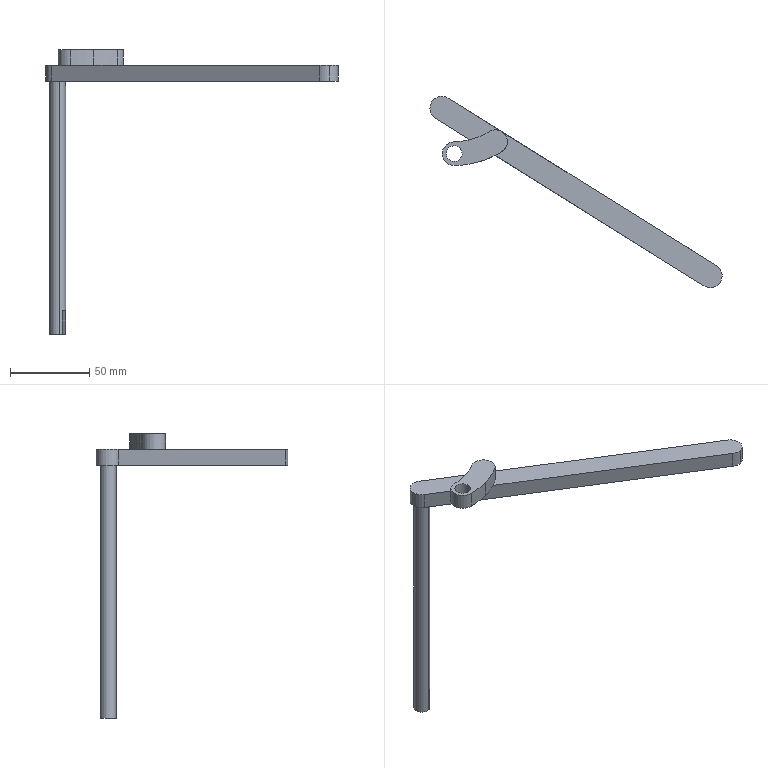Component | SolidWorks | DRocker(Right)-1 | 1 solid | 31 faces | box 184.66 x 120.91 x 180 mm | volume 48377 mm3 | cylinder 17 | plane 14 | commonest cylinder face diameters 15 x5 7 x4 10 x4 120 x2 90 x2
build123d program:
from build123d import *

# Parameters (mm, degrees)
BOSS_EXTRUDE1_DEPTH = 10
SKETCH1_3_R         = 5
BOSS_EXTRUDE2_DEPTH = 160
BOSS_EXTRUDE3_START = 10
SKETCH1_4_2_R       = 5
BOSS_EXTRUDE3_DEPTH = 10
SKETCH2_R           = 5
BOSS_EXTRUDE4_DEPTH = 10
CUT_EXTRUDE1_DEPTH  = 15
SKETCH4_R           = 3.5
CUT_EXTRUDE2_DEPTH  = 10


with BuildPart() as part:
    # Sketch1_4 → Boss-Extrude1 (new body)
    with BuildSketch(Plane.XY):
        with BuildLine():
            Line((-210.677, 89.978), (-358.098, -45.177))
            ThreePointArc((-358.098, -45.177), (-368.695, -44.717), (-368.235, -34.121))
            Line((-368.235, -34.121), (-220.814, 101.035))
            ThreePointArc((-220.814, 101.035), (-210.217, 100.575), (-210.677, 89.978))
        make_face()
    extrude(amount=BOSS_EXTRUDE1_DEPTH)

    # Sketch1_3 → Boss-Extrude2 (add)
    with BuildSketch(Plane.XY):
        with Locations((-215.746, 95.507)):
            Circle(SKETCH1_3_R)
    extrude(amount=-BOSS_EXTRUDE2_DEPTH)

    # Sketch1_4 2 → Boss-Extrude3 (add)
    with BuildSketch(Plane.XY.offset(BOSS_EXTRUDE3_START)):
        with Locations((-245.23, 68.476)):
            Circle(SKETCH1_4_2_R)
    extrude(amount=BOSS_EXTRUDE3_DEPTH)

    # Sketch2 → Boss-Extrude4 (add)
    with BuildSketch(Plane.XY.offset(10)):
        with BuildLine():
            ThreePointArc((-252.451, 66.449), (-254.679, 81.953), (-252.818, 97.505))
            ThreePointArc((-252.818, 97.505), (-243.695, 102.917), (-238.284, 93.794))
            ThreePointArc((-238.284, 93.794), (-239.68, 82.13), (-238.009, 70.502))
            ThreePointArc((-238.009, 70.502), (-243.203, 61.255), (-252.451, 66.449))
        make_face()
        with Locations(Location((-245.551, 95.65, 0), (0, 0, 180))):
            Circle(SKETCH2_R, mode=Mode.SUBTRACT)
    extrude(amount=BOSS_EXTRUDE4_DEPTH)

    # Sketch3 → Cut-Extrude1 (cut)
    with BuildSketch(Plane(origin=(0, 0, -160), x_dir=(-1, 0, 0), z_dir=(0, 0, -1))):
        Polygon((214.394, 94.033), (221.765, 87.275), (224.468, 90.223), (217.097, 96.981), align=None)
    extrude(amount=-CUT_EXTRUDE1_DEPTH, mode=Mode.SUBTRACT)

    # Sketch4 → Cut-Extrude2 (cut)
    with BuildSketch(Plane(origin=(-141.032, 153.83, 0), x_dir=(0.7371, 0.6758, 0), z_dir=(0.6758, -0.7371, 0))):
        with Locations((-274.486, 5)):
            Circle(SKETCH4_R)
        with Locations((-154.486, 5)):
            Circle(SKETCH4_R)
    extrude(amount=-CUT_EXTRUDE2_DEPTH, mode=Mode.SUBTRACT)


solid = part.part

# Placed as in the assembly
solid = solid.moved(Location((205.792, 280.96, 117.182), (0, 0, 105.511)))
STEP:
#1=COLOUR_RGB('',0.7922,0.8196,0.9333);
#2=FILL_AREA_STYLE_COLOUR('',#1);
#3=FILL_AREA_STYLE('',(#2));
#4=SURFACE_STYLE_FILL_AREA(#3);
#5=SURFACE_SIDE_STYLE('',(#4));
#6=SURFACE_STYLE_USAGE(.BOTH.,#5);
#7=PRESENTATION_STYLE_ASSIGNMENT((#6));
#8=CARTESIAN_POINT('',(12.827,-2.038,4.81));
#9=VERTEX_POINT('',#8);
#10=CARTESIAN_POINT('',(12.593,-1.892,4.81));
#11=VERTEX_POINT('',#10);
#12=CARTESIAN_POINT('',(12.71,-1.965,4.81));
#13=DIRECTION('',(0.5295,0.8483,-0.));
#14=DIRECTION('',(-0.8483,0.5295,0.));
#15=AXIS2_PLACEMENT_3D('',#12,#13,#14);
#16=CIRCLE('',#15,0.1378);
#17=EDGE_CURVE('',#9,#11,#16,.T.);
#18=ORIENTED_EDGE('',*,*,#17,.F.);
#19=CARTESIAN_POINT('',(13.035,-1.704,4.81));
#20=VERTEX_POINT('',#19);
#21=CARTESIAN_POINT('',(12.827,-2.038,4.81));
#22=DIRECTION('',(0.5295,0.8483,-0.));
#23=VECTOR('',#22,39.37);
#24=LINE('',#21,#23);
#25=EDGE_CURVE('',#9,#20,#24,.T.);
#26=ORIENTED_EDGE('',*,*,#25,.T.);
#27=CARTESIAN_POINT('',(12.801,-1.558,4.81));
#28=VERTEX_POINT('',#27);
#29=CARTESIAN_POINT('',(12.918,-1.631,4.81));
#30=DIRECTION('',(0.5295,0.8483,-0.));
#31=DIRECTION('',(-0.8483,0.5295,0.));
#32=AXIS2_PLACEMENT_3D('',#29,#30,#31);
#33=CIRCLE('',#32,0.1378);
#34=EDGE_CURVE('',#20,#28,#33,.T.);
#35=ORIENTED_EDGE('',*,*,#34,.T.);
#36=CARTESIAN_POINT('',(12.593,-1.892,4.81));
#37=DIRECTION('',(0.5295,0.8483,-0.));
#38=VECTOR('',#37,39.37);
#39=LINE('',#36,#38);
#40=EDGE_CURVE('',#11,#28,#39,.T.);
#41=ORIENTED_EDGE('',*,*,#40,.F.);
#42=EDGE_LOOP('',(#18,#26,#35,#41));
#43=FACE_OUTER_BOUND('',#42,.T.);
#44=CARTESIAN_POINT('',(12.71,-1.965,4.81));
#45=DIRECTION('',(0.5295,0.8483,-0.));
#46=DIRECTION('',(-0.8483,0.5295,0.));
#47=AXIS2_PLACEMENT_3D('',#44,#45,#46);
#48=CYLINDRICAL_SURFACE('',#47,0.1378);
#49=ADVANCED_FACE('',(#43),#48,.F.);
#50=CARTESIAN_POINT('',(8.819,0.464,4.81));
#51=VERTEX_POINT('',#50);
#52=CARTESIAN_POINT('',(8.585,0.6099,4.81));
#53=VERTEX_POINT('',#52);
#54=CARTESIAN_POINT('',(8.702,0.5369,4.81));
#55=DIRECTION('',(0.5295,0.8483,-0.));
#56=DIRECTION('',(-0.8483,0.5295,0.));
#57=AXIS2_PLACEMENT_3D('',#54,#55,#56);
#58=CIRCLE('',#57,0.1378);
#59=EDGE_CURVE('',#51,#53,#58,.T.);
#60=ORIENTED_EDGE('',*,*,#59,.F.);
#61=CARTESIAN_POINT('',(9.027,0.7979,4.81));
#62=VERTEX_POINT('',#61);
#63=CARTESIAN_POINT('',(8.819,0.464,4.81));
#64=DIRECTION('',(0.5295,0.8483,-0.));
#65=VECTOR('',#64,39.37);
#66=LINE('',#63,#65);
#67=EDGE_CURVE('',#51,#62,#66,.T.);
#68=ORIENTED_EDGE('',*,*,#67,.T.);
#69=CARTESIAN_POINT('',(8.794,0.9439,4.81));
#70=VERTEX_POINT('',#69);
#71=CARTESIAN_POINT('',(8.911,0.8709,4.81));
#72=DIRECTION('',(0.5295,0.8483,-0.));
#73=DIRECTION('',(-0.8483,0.5295,0.));
#74=AXIS2_PLACEMENT_3D('',#71,#72,#73);
#75=CIRCLE('',#74,0.1378);
#76=EDGE_CURVE('',#62,#70,#75,.T.);
#77=ORIENTED_EDGE('',*,*,#76,.T.);
#78=CARTESIAN_POINT('',(8.585,0.6099,4.81));
#79=DIRECTION('',(0.5295,0.8483,-0.));
#80=VECTOR('',#79,39.37);
#81=LINE('',#78,#80);
#82=EDGE_CURVE('',#53,#70,#81,.T.);
#83=ORIENTED_EDGE('',*,*,#82,.F.);
#84=EDGE_LOOP('',(#60,#68,#77,#83));
#85=FACE_OUTER_BOUND('',#84,.T.);
#86=CARTESIAN_POINT('',(8.702,0.5369,4.81));
#87=DIRECTION('',(0.5295,0.8483,-0.));
#88=DIRECTION('',(-0.8483,0.5295,0.));
#89=AXIS2_PLACEMENT_3D('',#86,#87,#88);
#90=CYLINDRICAL_SURFACE('',#89,0.1378);
#91=ADVANCED_FACE('',(#85),#90,.F.);
#92=CARTESIAN_POINT('',(7.111,0.5494,5.401));
#93=VERTEX_POINT('',#92);
#94=CARTESIAN_POINT('',(7.006,0.9288,5.401));
#95=VERTEX_POINT('',#94);
#96=CARTESIAN_POINT('',(7.059,0.7391,5.401));
#97=DIRECTION('',(-0.,0.,1.));
#98=DIRECTION('',(0.2674,-0.9636,0.));
#99=AXIS2_PLACEMENT_3D('',#96,#97,#98);
#100=CIRCLE('',#99,0.1969);
#101=EDGE_CURVE('',#93,#95,#100,.T.);
#102=ORIENTED_EDGE('',*,*,#101,.T.);
#103=CARTESIAN_POINT('',(7.006,0.9288,5.007));
#104=VERTEX_POINT('',#103);
#105=CARTESIAN_POINT('',(7.006,0.9288,5.401));
#106=DIRECTION('',(0.,-0.,-1.));
#107=VECTOR('',#106,39.37);
#108=LINE('',#105,#107);
#109=EDGE_CURVE('',#95,#104,#108,.T.);
#110=ORIENTED_EDGE('',*,*,#109,.T.);
#111=CARTESIAN_POINT('',(7.111,0.5494,5.007));
#112=VERTEX_POINT('',#111);
#113=CARTESIAN_POINT('',(7.059,0.7391,5.007));
#114=DIRECTION('',(-0.,0.,1.));
#115=DIRECTION('',(0.2674,-0.9636,0.));
#116=AXIS2_PLACEMENT_3D('',#113,#114,#115);
#117=CIRCLE('',#116,0.1969);
#118=EDGE_CURVE('',#112,#104,#117,.T.);
#119=ORIENTED_EDGE('',*,*,#118,.F.);
#120=CARTESIAN_POINT('',(7.111,0.5494,5.401));
#121=DIRECTION('',(0.,-0.,-1.));
#122=VECTOR('',#121,39.37);
#123=LINE('',#120,#122);
#124=EDGE_CURVE('',#93,#112,#123,.T.);
#125=ORIENTED_EDGE('',*,*,#124,.F.);
#126=EDGE_LOOP('',(#102,#110,#119,#125));
#127=FACE_OUTER_BOUND('',#126,.T.);
#128=CARTESIAN_POINT('',(7.059,0.7391,5.401));
#129=DIRECTION('',(0.,-0.,-1.));
#130=DIRECTION('',(0.2674,-0.9636,0.));
#131=AXIS2_PLACEMENT_3D('',#128,#129,#130);
#132=CYLINDRICAL_SURFACE('',#131,0.1969);
#133=ADVANCED_FACE('',(#127),#132,.F.);
#134=CARTESIAN_POINT('',(7.648,0.5294,5.401));
#135=VERTEX_POINT('',#134);
#136=CARTESIAN_POINT('',(8.239,0.7848,5.401));
#137=VERTEX_POINT('',#136);
#138=CARTESIAN_POINT('',(7.016,2.806,5.401));
#139=DIRECTION('',(-0.,0.,1.));
#140=DIRECTION('',(0.2674,-0.9636,0.));
#141=AXIS2_PLACEMENT_3D('',#138,#139,#140);
#142=CIRCLE('',#141,2.362);
#143=EDGE_CURVE('',#135,#137,#142,.T.);
#144=ORIENTED_EDGE('',*,*,#143,.F.);
#145=CARTESIAN_POINT('',(7.648,0.5294,5.007));
#146=VERTEX_POINT('',#145);
#147=CARTESIAN_POINT('',(7.648,0.5294,5.401));
#148=DIRECTION('',(0.,-0.,-1.));
#149=VECTOR('',#148,39.37);
#150=LINE('',#147,#149);
#151=EDGE_CURVE('',#135,#146,#150,.T.);
#152=ORIENTED_EDGE('',*,*,#151,.T.);
#153=CARTESIAN_POINT('',(8.077,0.6951,5.007));
#154=VERTEX_POINT('',#153);
#155=CARTESIAN_POINT('',(7.016,2.806,5.007));
#156=DIRECTION('',(-0.,0.,1.));
#157=DIRECTION('',(0.2674,-0.9636,0.));
#158=AXIS2_PLACEMENT_3D('',#155,#156,#157);
#159=CIRCLE('',#158,2.362);
#160=EDGE_CURVE('',#146,#154,#159,.T.);
#161=ORIENTED_EDGE('',*,*,#160,.T.);
#162=CARTESIAN_POINT('',(8.239,0.7848,5.007));
#163=VERTEX_POINT('',#162);
#164=CARTESIAN_POINT('',(7.016,2.806,5.007));
#165=DIRECTION('',(-0.,0.,1.));
#166=DIRECTION('',(0.2674,-0.9636,0.));
#167=AXIS2_PLACEMENT_3D('',#164,#165,#166);
#168=CIRCLE('',#167,2.362);
#169=EDGE_CURVE('',#154,#163,#168,.T.);
#170=ORIENTED_EDGE('',*,*,#169,.T.);
#171=CARTESIAN_POINT('',(8.239,0.7848,5.401));
#172=DIRECTION('',(0.,-0.,-1.));
#173=VECTOR('',#172,39.37);
#174=LINE('',#171,#173);
#175=EDGE_CURVE('',#137,#163,#174,.T.);
#176=ORIENTED_EDGE('',*,*,#175,.F.);
#177=EDGE_LOOP('',(#144,#152,#161,#170,#176));
#178=FACE_OUTER_BOUND('',#177,.T.);
#179=CARTESIAN_POINT('',(7.016,2.806,5.401));
#180=DIRECTION('',(0.,-0.,-1.));
#181=DIRECTION('',(0.2674,-0.9636,0.));
#182=AXIS2_PLACEMENT_3D('',#179,#180,#181);
#183=CYLINDRICAL_SURFACE('',#182,2.362);
#184=ADVANCED_FACE('',(#178),#183,.T.);
#185=CARTESIAN_POINT('',(7.49,1.098,5.401));
#186=VERTEX_POINT('',#185);
#187=CARTESIAN_POINT('',(7.053,1.034,5.401));
#188=VERTEX_POINT('',#187);
#189=CARTESIAN_POINT('',(7.016,2.806,5.401));
#190=DIRECTION('',(0.,-0.,-1.));
#191=DIRECTION('',(0.2674,-0.9636,0.));
#192=AXIS2_PLACEMENT_3D('',#189,#190,#191);
#193=CIRCLE('',#192,1.772);
#194=EDGE_CURVE('',#186,#188,#193,.T.);
#195=ORIENTED_EDGE('',*,*,#194,.F.);
#196=CARTESIAN_POINT('',(7.49,1.098,5.007));
#197=VERTEX_POINT('',#196);
#198=CARTESIAN_POINT('',(7.49,1.098,5.401));
#199=DIRECTION('',(0.,-0.,-1.));
#200=VECTOR('',#199,39.37);
#201=LINE('',#198,#200);
#202=EDGE_CURVE('',#186,#197,#201,.T.);
#203=ORIENTED_EDGE('',*,*,#202,.T.);
#204=CARTESIAN_POINT('',(7.448,1.088,5.007));
#205=VERTEX_POINT('',#204);
#206=CARTESIAN_POINT('',(7.016,2.806,5.007));
#207=DIRECTION('',(0.,-0.,-1.));
#208=DIRECTION('',(0.2674,-0.9636,0.));
#209=AXIS2_PLACEMENT_3D('',#206,#207,#208);
#210=CIRCLE('',#209,1.772);
#211=EDGE_CURVE('',#197,#205,#210,.T.);
#212=ORIENTED_EDGE('',*,*,#211,.T.);
#213=CARTESIAN_POINT('',(7.053,1.034,5.007));
#214=VERTEX_POINT('',#213);
#215=CARTESIAN_POINT('',(7.016,2.806,5.007));
#216=DIRECTION('',(0.,-0.,-1.));
#217=DIRECTION('',(0.2674,-0.9636,0.));
#218=AXIS2_PLACEMENT_3D('',#215,#216,#217);
#219=CIRCLE('',#218,1.772);
#220=EDGE_CURVE('',#205,#214,#219,.T.);
#221=ORIENTED_EDGE('',*,*,#220,.T.);
#222=CARTESIAN_POINT('',(7.053,1.034,5.401));
#223=DIRECTION('',(0.,-0.,-1.));
#224=VECTOR('',#223,39.37);
#225=LINE('',#222,#224);
#226=EDGE_CURVE('',#188,#214,#225,.T.);
#227=ORIENTED_EDGE('',*,*,#226,.F.);
#228=EDGE_LOOP('',(#195,#203,#212,#221,#227));
#229=FACE_OUTER_BOUND('',#228,.T.);
#230=CARTESIAN_POINT('',(7.016,2.806,5.401));
#231=DIRECTION('',(0.,-0.,-1.));
#232=DIRECTION('',(0.2674,-0.9636,0.));
#233=AXIS2_PLACEMENT_3D('',#230,#231,#232);
#234=CYLINDRICAL_SURFACE('',#233,1.772);
#235=ADVANCED_FACE('',(#229),#234,.F.);
#236=CARTESIAN_POINT('',(6.698,2.061,-1.686));
#237=VERTEX_POINT('',#236);
#238=CARTESIAN_POINT('',(6.803,1.682,-1.686));
#239=VERTEX_POINT('',#238);
#240=CARTESIAN_POINT('',(6.75,1.871,-1.686));
#241=DIRECTION('',(-0.,0.,1.));
#242=DIRECTION('',(-0.2674,0.9636,0.));
#243=AXIS2_PLACEMENT_3D('',#240,#241,#242);
#244=CIRCLE('',#243,0.1969);
#245=EDGE_CURVE('',#237,#239,#244,.T.);
#246=ORIENTED_EDGE('',*,*,#245,.T.);
#247=CARTESIAN_POINT('',(6.803,1.682,4.613));
#248=VERTEX_POINT('',#247);
#249=CARTESIAN_POINT('',(6.803,1.682,-1.686));
#250=DIRECTION('',(-0.,0.,1.));
#251=VECTOR('',#250,39.37);
#252=LINE('',#249,#251);
#253=EDGE_CURVE('',#239,#248,#252,.T.);
#254=ORIENTED_EDGE('',*,*,#253,.T.);
#255=CARTESIAN_POINT('',(6.698,2.061,4.613));
#256=VERTEX_POINT('',#255);
#257=CARTESIAN_POINT('',(6.75,1.871,4.613));
#258=DIRECTION('',(-0.,0.,1.));
#259=DIRECTION('',(-0.2674,0.9636,0.));
#260=AXIS2_PLACEMENT_3D('',#257,#258,#259);
#261=CIRCLE('',#260,0.1969);
#262=EDGE_CURVE('',#256,#248,#261,.T.);
#263=ORIENTED_EDGE('',*,*,#262,.F.);
#264=CARTESIAN_POINT('',(6.698,2.061,-1.686));
#265=DIRECTION('',(-0.,0.,1.));
#266=VECTOR('',#265,39.37);
#267=LINE('',#264,#266);
#268=EDGE_CURVE('',#237,#256,#267,.T.);
#269=ORIENTED_EDGE('',*,*,#268,.F.);
#270=EDGE_LOOP('',(#246,#254,#263,#269));
#271=FACE_OUTER_BOUND('',#270,.T.);
#272=CARTESIAN_POINT('',(6.75,1.871,-1.686));
#273=DIRECTION('',(-0.,0.,1.));
#274=DIRECTION('',(-0.2674,0.9636,0.));
#275=AXIS2_PLACEMENT_3D('',#272,#273,#274);
#276=CYLINDRICAL_SURFACE('',#275,0.1969);
#277=ADVANCED_FACE('',(#271),#276,.T.);
#278=CARTESIAN_POINT('',(13.509,-2.583,5.007));
#279=VERTEX_POINT('',#278);
#280=CARTESIAN_POINT('',(13.586,-2.048,5.007));
#281=VERTEX_POINT('',#280);
#282=CARTESIAN_POINT('',(13.43,-2.298,5.007));
#283=DIRECTION('',(-0.,0.,1.));
#284=DIRECTION('',(-0.2674,0.9636,0.));
#285=AXIS2_PLACEMENT_3D('',#282,#283,#284);
#286=CIRCLE('',#285,0.2953);
#287=EDGE_CURVE('',#279,#281,#286,.T.);
#288=ORIENTED_EDGE('',*,*,#287,.F.);
#289=CARTESIAN_POINT('',(13.509,-2.583,4.613));
#290=VERTEX_POINT('',#289);
#291=CARTESIAN_POINT('',(13.509,-2.583,5.007));
#292=DIRECTION('',(0.,-0.,-1.));
#293=VECTOR('',#292,39.37);
#294=LINE('',#291,#293);
#295=EDGE_CURVE('',#279,#290,#294,.T.);
#296=ORIENTED_EDGE('',*,*,#295,.T.);
#297=CARTESIAN_POINT('',(13.586,-2.048,4.613));
#298=VERTEX_POINT('',#297);
#299=CARTESIAN_POINT('',(13.43,-2.298,4.613));
#300=DIRECTION('',(-0.,0.,1.));
#301=DIRECTION('',(-0.2674,0.9636,0.));
#302=AXIS2_PLACEMENT_3D('',#299,#300,#301);
#303=CIRCLE('',#302,0.2953);
#304=EDGE_CURVE('',#290,#298,#303,.T.);
#305=ORIENTED_EDGE('',*,*,#304,.T.);
#306=CARTESIAN_POINT('',(13.586,-2.048,5.007));
#307=DIRECTION('',(0.,-0.,-1.));
#308=VECTOR('',#307,39.37);
#309=LINE('',#306,#308);
#310=EDGE_CURVE('',#281,#298,#309,.T.);
#311=ORIENTED_EDGE('',*,*,#310,.F.);
#312=EDGE_LOOP('',(#288,#296,#305,#311));
#313=FACE_OUTER_BOUND('',#312,.T.);
#314=CARTESIAN_POINT('',(13.43,-2.298,5.007));
#315=DIRECTION('',(0.,-0.,-1.));
#316=DIRECTION('',(0.2674,-0.9636,0.));
#317=AXIS2_PLACEMENT_3D('',#314,#315,#316);
#318=CYLINDRICAL_SURFACE('',#317,0.2953);
#319=ADVANCED_FACE('',(#313),#318,.T.);
#320=CARTESIAN_POINT('',(6.594,1.621,5.007));
#321=VERTEX_POINT('',#320);
#322=CARTESIAN_POINT('',(3.438,3.591,5.007));
#323=DIRECTION('',(0.8483,-0.5295,0.));
#324=VECTOR('',#323,39.37);
#325=LINE('',#322,#324);
#326=EDGE_CURVE('',#321,#205,#325,.T.);
#327=ORIENTED_EDGE('',*,*,#326,.T.);
#328=ORIENTED_EDGE('',*,*,#211,.F.);
#329=CARTESIAN_POINT('',(7.933,1.29,5.007));
#330=VERTEX_POINT('',#329);
#331=CARTESIAN_POINT('',(7.016,2.806,5.007));
#332=DIRECTION('',(0.,-0.,-1.));
#333=DIRECTION('',(0.2674,-0.9636,0.));
#334=AXIS2_PLACEMENT_3D('',#331,#332,#333);
#335=CIRCLE('',#334,1.772);
#336=EDGE_CURVE('',#330,#197,#335,.T.);
#337=ORIENTED_EDGE('',*,*,#336,.F.);
#338=CARTESIAN_POINT('',(8.243,1.288,5.007));
#339=VERTEX_POINT('',#338);
#340=CARTESIAN_POINT('',(8.086,1.037,5.007));
#341=DIRECTION('',(-0.,0.,1.));
#342=DIRECTION('',(0.2674,-0.9636,0.));
#343=AXIS2_PLACEMENT_3D('',#340,#341,#342);
#344=CIRCLE('',#343,0.2953);
#345=EDGE_CURVE('',#339,#330,#344,.T.);
#346=ORIENTED_EDGE('',*,*,#345,.F.);
#347=CARTESIAN_POINT('',(6.907,2.122,5.007));
#348=VERTEX_POINT('',#347);
#349=CARTESIAN_POINT('',(3.751,4.092,5.007));
#350=DIRECTION('',(0.8483,-0.5295,0.));
#351=VECTOR('',#350,39.37);
#352=LINE('',#349,#351);
#353=EDGE_CURVE('',#348,#339,#352,.T.);
#354=ORIENTED_EDGE('',*,*,#353,.F.);
#355=CARTESIAN_POINT('',(6.75,1.871,5.007));
#356=DIRECTION('',(-0.,0.,1.));
#357=DIRECTION('',(-0.2674,0.9636,0.));
#358=AXIS2_PLACEMENT_3D('',#355,#356,#357);
#359=CIRCLE('',#358,0.2953);
#360=EDGE_CURVE('',#348,#321,#359,.T.);
#361=ORIENTED_EDGE('',*,*,#360,.T.);
#362=EDGE_LOOP('',(#327,#328,#337,#346,#354,#361));
#363=FACE_OUTER_BOUND('',#362,.T.);
#364=CARTESIAN_POINT('',(8.102,11.061,5.007));
#365=DIRECTION('',(-0.,0.,1.));
#366=DIRECTION('',(-0.2674,0.9636,-0.));
#367=AXIS2_PLACEMENT_3D('',#364,#365,#366);
#368=PLANE('',#367);
#369=ADVANCED_FACE('',(#363),#368,.T.);
#370=CARTESIAN_POINT('',(6.594,1.621,4.613));
#371=VERTEX_POINT('',#370);
#372=CARTESIAN_POINT('',(13.273,-2.549,4.613));
#373=VERTEX_POINT('',#372);
#374=CARTESIAN_POINT('',(3.438,3.591,4.613));
#375=DIRECTION('',(0.8483,-0.5295,0.));
#376=VECTOR('',#375,39.37);
#377=LINE('',#374,#376);
#378=EDGE_CURVE('',#371,#373,#377,.T.);
#379=ORIENTED_EDGE('',*,*,#378,.T.);
#380=CARTESIAN_POINT('',(13.273,-2.549,5.007));
#381=VERTEX_POINT('',#380);
#382=CARTESIAN_POINT('',(13.273,-2.549,5.007));
#383=DIRECTION('',(0.,-0.,-1.));
#384=VECTOR('',#383,39.37);
#385=LINE('',#382,#384);
#386=EDGE_CURVE('',#381,#373,#385,.T.);
#387=ORIENTED_EDGE('',*,*,#386,.F.);
#388=CARTESIAN_POINT('',(3.438,3.591,5.007));
#389=DIRECTION('',(0.8483,-0.5295,0.));
#390=VECTOR('',#389,39.37);
#391=LINE('',#388,#390);
#392=EDGE_CURVE('',#154,#381,#391,.T.);
#393=ORIENTED_EDGE('',*,*,#392,.F.);
#394=CARTESIAN_POINT('',(3.438,3.591,5.007));
#395=DIRECTION('',(-0.8483,0.5295,-0.));
#396=VECTOR('',#395,39.37);
#397=LINE('',#394,#396);
#398=EDGE_CURVE('',#154,#205,#397,.T.);
#399=ORIENTED_EDGE('',*,*,#398,.T.);
#400=ORIENTED_EDGE('',*,*,#326,.F.);
#401=CARTESIAN_POINT('',(6.594,1.621,5.007));
#402=DIRECTION('',(0.,-0.,-1.));
#403=VECTOR('',#402,39.37);
#404=LINE('',#401,#403);
#405=EDGE_CURVE('',#321,#371,#404,.T.);
#406=ORIENTED_EDGE('',*,*,#405,.T.);
#407=EDGE_LOOP('',(#379,#387,#393,#399,#400,#406));
#408=FACE_OUTER_BOUND('',#407,.T.);
#409=CARTESIAN_POINT('',(3.438,3.591,5.007));
#410=DIRECTION('',(0.5295,0.8483,-0.));
#411=DIRECTION('',(-0.8483,0.5295,-0.));
#412=AXIS2_PLACEMENT_3D('',#409,#410,#411);
#413=PLANE('',#412);
#414=ADVANCED_FACE('',(#408),#413,.F.);
#415=ORIENTED_EDGE('',*,*,#295,.F.);
#416=CARTESIAN_POINT('',(13.43,-2.298,5.007));
#417=DIRECTION('',(-0.,0.,1.));
#418=DIRECTION('',(-0.2674,0.9636,0.));
#419=AXIS2_PLACEMENT_3D('',#416,#417,#418);
#420=CIRCLE('',#419,0.2953);
#421=EDGE_CURVE('',#381,#279,#420,.T.);
#422=ORIENTED_EDGE('',*,*,#421,.F.);
#423=ORIENTED_EDGE('',*,*,#386,.T.);
#424=CARTESIAN_POINT('',(13.43,-2.298,4.613));
#425=DIRECTION('',(-0.,0.,1.));
#426=DIRECTION('',(-0.2674,0.9636,0.));
#427=AXIS2_PLACEMENT_3D('',#424,#425,#426);
#428=CIRCLE('',#427,0.2953);
#429=EDGE_CURVE('',#373,#290,#428,.T.);
#430=ORIENTED_EDGE('',*,*,#429,.T.);
#431=EDGE_LOOP('',(#415,#422,#423,#430));
#432=FACE_OUTER_BOUND('',#431,.T.);
#433=CARTESIAN_POINT('',(13.43,-2.298,5.007));
#434=DIRECTION('',(0.,-0.,-1.));
#435=DIRECTION('',(0.2674,-0.9636,0.));
#436=AXIS2_PLACEMENT_3D('',#433,#434,#435);
#437=CYLINDRICAL_SURFACE('',#436,0.2953);
#438=ADVANCED_FACE('',(#432),#437,.T.);
#439=CARTESIAN_POINT('',(12.918,-1.631,4.81));
#440=DIRECTION('',(0.5295,0.8483,-0.));
#441=DIRECTION('',(-0.8483,0.5295,0.));
#442=AXIS2_PLACEMENT_3D('',#439,#440,#441);
#443=CIRCLE('',#442,0.1378);
#444=EDGE_CURVE('',#28,#20,#443,.T.);
#445=ORIENTED_EDGE('',*,*,#444,.F.);
#446=ORIENTED_EDGE('',*,*,#34,.F.);
#447=EDGE_LOOP('',(#445,#446));
#448=FACE_BOUND('',#447,.T.);
#449=CARTESIAN_POINT('',(8.911,0.8709,4.81));
#450=DIRECTION('',(0.5295,0.8483,-0.));
#451=DIRECTION('',(-0.8483,0.5295,0.));
#452=AXIS2_PLACEMENT_3D('',#449,#450,#451);
#453=CIRCLE('',#452,0.1378);
#454=EDGE_CURVE('',#70,#62,#453,.T.);
#455=ORIENTED_EDGE('',*,*,#454,.F.);
#456=ORIENTED_EDGE('',*,*,#76,.F.);
#457=EDGE_LOOP('',(#455,#456));
#458=FACE_BOUND('',#457,.T.);
#459=CARTESIAN_POINT('',(6.907,2.122,4.613));
#460=VERTEX_POINT('',#459);
#461=CARTESIAN_POINT('',(3.751,4.092,4.613));
#462=DIRECTION('',(0.8483,-0.5295,0.));
#463=VECTOR('',#462,39.37);
#464=LINE('',#461,#463);
#465=EDGE_CURVE('',#460,#298,#464,.T.);
#466=ORIENTED_EDGE('',*,*,#465,.F.);
#467=CARTESIAN_POINT('',(6.907,2.122,5.007));
#468=DIRECTION('',(0.,-0.,-1.));
#469=VECTOR('',#468,39.37);
#470=LINE('',#467,#469);
#471=EDGE_CURVE('',#348,#460,#470,.T.);
#472=ORIENTED_EDGE('',*,*,#471,.F.);
#473=ORIENTED_EDGE('',*,*,#353,.T.);
#474=CARTESIAN_POINT('',(3.751,4.092,5.007));
#475=DIRECTION('',(0.8483,-0.5295,0.));
#476=VECTOR('',#475,39.37);
#477=LINE('',#474,#476);
#478=EDGE_CURVE('',#339,#281,#477,.T.);
#479=ORIENTED_EDGE('',*,*,#478,.T.);
#480=ORIENTED_EDGE('',*,*,#310,.T.);
#481=EDGE_LOOP('',(#466,#472,#473,#479,#480));
#482=FACE_OUTER_BOUND('',#481,.T.);
#483=CARTESIAN_POINT('',(3.751,4.092,5.007));
#484=DIRECTION('',(0.5295,0.8483,-0.));
#485=DIRECTION('',(-0.8483,0.5295,-0.));
#486=AXIS2_PLACEMENT_3D('',#483,#484,#485);
#487=PLANE('',#486);
#488=ADVANCED_FACE('',(#448,#458,#482),#487,.T.);
#489=CARTESIAN_POINT('',(6.75,1.871,4.613));
#490=DIRECTION('',(-0.,0.,1.));
#491=DIRECTION('',(-0.2674,0.9636,0.));
#492=AXIS2_PLACEMENT_3D('',#489,#490,#491);
#493=CIRCLE('',#492,0.2953);
#494=EDGE_CURVE('',#460,#371,#493,.T.);
#495=ORIENTED_EDGE('',*,*,#494,.T.);
#496=ORIENTED_EDGE('',*,*,#405,.F.);
#497=ORIENTED_EDGE('',*,*,#360,.F.);
#498=ORIENTED_EDGE('',*,*,#471,.T.);
#499=EDGE_LOOP('',(#495,#496,#497,#498));
#500=FACE_OUTER_BOUND('',#499,.T.);
#501=CARTESIAN_POINT('',(6.75,1.871,5.007));
#502=DIRECTION('',(0.,-0.,-1.));
#503=DIRECTION('',(0.2674,-0.9636,0.));
#504=AXIS2_PLACEMENT_3D('',#501,#502,#503);
#505=CYLINDRICAL_SURFACE('',#504,0.2953);
#506=ADVANCED_FACE('',(#500),#505,.T.);
#507=ORIENTED_EDGE('',*,*,#478,.F.);
#508=CARTESIAN_POINT('',(8.086,1.037,5.007));
#509=DIRECTION('',(-0.,0.,1.));
#510=DIRECTION('',(0.2674,-0.9636,0.));
#511=AXIS2_PLACEMENT_3D('',#508,#509,#510);
#512=CIRCLE('',#511,0.2953);
#513=EDGE_CURVE('',#163,#339,#512,.T.);
#514=ORIENTED_EDGE('',*,*,#513,.F.);
#515=ORIENTED_EDGE('',*,*,#169,.F.);
#516=ORIENTED_EDGE('',*,*,#392,.T.);
#517=ORIENTED_EDGE('',*,*,#421,.T.);
#518=ORIENTED_EDGE('',*,*,#287,.T.);
#519=EDGE_LOOP('',(#507,#514,#515,#516,#517,#518));
#520=FACE_OUTER_BOUND('',#519,.T.);
#521=CARTESIAN_POINT('',(8.102,11.061,5.007));
#522=DIRECTION('',(-0.,0.,1.));
#523=DIRECTION('',(-0.2674,0.9636,-0.));
#524=AXIS2_PLACEMENT_3D('',#521,#522,#523);
#525=PLANE('',#524);
#526=ADVANCED_FACE('',(#520),#525,.T.);
#527=ORIENTED_EDGE('',*,*,#262,.T.);
#528=CARTESIAN_POINT('',(6.75,1.871,4.613));
#529=DIRECTION('',(-0.,0.,1.));
#530=DIRECTION('',(-0.2674,0.9636,0.));
#531=AXIS2_PLACEMENT_3D('',#528,#529,#530);
#532=CIRCLE('',#531,0.1969);
#533=EDGE_CURVE('',#248,#256,#532,.T.);
#534=ORIENTED_EDGE('',*,*,#533,.T.);
#535=EDGE_LOOP('',(#527,#534));
#536=FACE_BOUND('',#535,.T.);
#537=ORIENTED_EDGE('',*,*,#378,.F.);
#538=ORIENTED_EDGE('',*,*,#494,.F.);
#539=ORIENTED_EDGE('',*,*,#465,.T.);
#540=ORIENTED_EDGE('',*,*,#304,.F.);
#541=ORIENTED_EDGE('',*,*,#429,.F.);
#542=EDGE_LOOP('',(#537,#538,#539,#540,#541));
#543=FACE_OUTER_BOUND('',#542,.T.);
#544=CARTESIAN_POINT('',(8.102,11.061,4.613));
#545=DIRECTION('',(-0.,0.,1.));
#546=DIRECTION('',(-0.2674,0.9636,-0.));
#547=AXIS2_PLACEMENT_3D('',#544,#545,#546);
#548=PLANE('',#547);
#549=ADVANCED_FACE('',(#536,#543),#548,.F.);
#550=ORIENTED_EDGE('',*,*,#253,.F.);
#551=CARTESIAN_POINT('',(6.862,1.709,-1.686));
#552=VERTEX_POINT('',#551);
#553=CARTESIAN_POINT('',(6.75,1.871,-1.686));
#554=DIRECTION('',(-0.,0.,1.));
#555=DIRECTION('',(-0.2674,0.9636,0.));
#556=AXIS2_PLACEMENT_3D('',#553,#554,#555);
#557=CIRCLE('',#556,0.1969);
#558=EDGE_CURVE('',#239,#552,#557,.T.);
#559=ORIENTED_EDGE('',*,*,#558,.T.);
#560=CARTESIAN_POINT('',(6.862,1.709,-1.095));
#561=VERTEX_POINT('',#560);
#562=CARTESIAN_POINT('',(6.862,1.709,-1.686));
#563=DIRECTION('',(0.,-0.,-1.));
#564=VECTOR('',#563,39.37);
#565=LINE('',#562,#564);
#566=EDGE_CURVE('',#561,#552,#565,.T.);
#567=ORIENTED_EDGE('',*,*,#566,.F.);
#568=CARTESIAN_POINT('',(6.945,1.843,-1.095));
#569=VERTEX_POINT('',#568);
#570=CARTESIAN_POINT('',(6.75,1.871,-1.095));
#571=DIRECTION('',(0.,-0.,-1.));
#572=DIRECTION('',(-0.2674,0.9636,0.));
#573=AXIS2_PLACEMENT_3D('',#570,#571,#572);
#574=CIRCLE('',#573,0.1969);
#575=EDGE_CURVE('',#569,#561,#574,.T.);
#576=ORIENTED_EDGE('',*,*,#575,.F.);
#577=CARTESIAN_POINT('',(6.945,1.843,-1.686));
#578=VERTEX_POINT('',#577);
#579=CARTESIAN_POINT('',(6.945,1.843,-1.686));
#580=DIRECTION('',(-0.,0.,1.));
#581=VECTOR('',#580,39.37);
#582=LINE('',#579,#581);
#583=EDGE_CURVE('',#578,#569,#582,.T.);
#584=ORIENTED_EDGE('',*,*,#583,.F.);
#585=CARTESIAN_POINT('',(6.75,1.871,-1.686));
#586=DIRECTION('',(-0.,0.,1.));
#587=DIRECTION('',(-0.2674,0.9636,0.));
#588=AXIS2_PLACEMENT_3D('',#585,#586,#587);
#589=CIRCLE('',#588,0.1969);
#590=EDGE_CURVE('',#578,#237,#589,.T.);
#591=ORIENTED_EDGE('',*,*,#590,.T.);
#592=ORIENTED_EDGE('',*,*,#268,.T.);
#593=ORIENTED_EDGE('',*,*,#533,.F.);
#594=EDGE_LOOP('',(#550,#559,#567,#576,#584,#591,#592,#593));
#595=FACE_OUTER_BOUND('',#594,.T.);
#596=CARTESIAN_POINT('',(6.75,1.871,-1.686));
#597=DIRECTION('',(-0.,0.,1.));
#598=DIRECTION('',(-0.2674,0.9636,0.));
#599=AXIS2_PLACEMENT_3D('',#596,#597,#598);
#600=CYLINDRICAL_SURFACE('',#599,0.1969);
#601=ADVANCED_FACE('',(#595),#600,.T.);
#602=CARTESIAN_POINT('',(6.709,1.805,-1.686));
#603=VERTEX_POINT('',#602);
#604=CARTESIAN_POINT('',(6.792,1.938,-1.686));
#605=VERTEX_POINT('',#604);
#606=CARTESIAN_POINT('',(6.792,1.938,-1.686));
#607=DIRECTION('',(0.5295,0.8483,-0.));
#608=VECTOR('',#607,39.37);
#609=LINE('',#606,#608);
#610=EDGE_CURVE('',#603,#605,#609,.T.);
#611=ORIENTED_EDGE('',*,*,#610,.F.);
#612=CARTESIAN_POINT('',(3.553,3.774,-1.686));
#613=DIRECTION('',(0.8483,-0.5295,0.));
#614=VECTOR('',#613,39.37);
#615=LINE('',#612,#614);
#616=EDGE_CURVE('',#603,#552,#615,.T.);
#617=ORIENTED_EDGE('',*,*,#616,.T.);
#618=ORIENTED_EDGE('',*,*,#558,.F.);
#619=ORIENTED_EDGE('',*,*,#245,.F.);
#620=ORIENTED_EDGE('',*,*,#590,.F.);
#621=CARTESIAN_POINT('',(6.792,1.938,-1.686));
#622=DIRECTION('',(0.8483,-0.5295,0.));
#623=VECTOR('',#622,39.37);
#624=LINE('',#621,#623);
#625=EDGE_CURVE('',#605,#578,#624,.T.);
#626=ORIENTED_EDGE('',*,*,#625,.F.);
#627=EDGE_LOOP('',(#611,#617,#618,#619,#620,#626));
#628=FACE_OUTER_BOUND('',#627,.T.);
#629=CARTESIAN_POINT('',(8.102,11.061,-1.686));
#630=DIRECTION('',(-0.,0.,1.));
#631=DIRECTION('',(-0.2674,0.9636,-0.));
#632=AXIS2_PLACEMENT_3D('',#629,#630,#631);
#633=PLANE('',#632);
#634=ADVANCED_FACE('',(#628),#633,.F.);
#635=ORIENTED_EDGE('',*,*,#398,.F.);
#636=ORIENTED_EDGE('',*,*,#160,.F.);
#637=CARTESIAN_POINT('',(7.065,0.4439,5.007));
#638=VERTEX_POINT('',#637);
#639=CARTESIAN_POINT('',(7.016,2.806,5.007));
#640=DIRECTION('',(-0.,0.,1.));
#641=DIRECTION('',(0.2674,-0.9636,0.));
#642=AXIS2_PLACEMENT_3D('',#639,#640,#641);
#643=CIRCLE('',#642,2.362);
#644=EDGE_CURVE('',#638,#146,#643,.T.);
#645=ORIENTED_EDGE('',*,*,#644,.F.);
#646=CARTESIAN_POINT('',(7.059,0.7391,5.007));
#647=DIRECTION('',(-0.,0.,1.));
#648=DIRECTION('',(0.2674,-0.9636,0.));
#649=AXIS2_PLACEMENT_3D('',#646,#647,#648);
#650=CIRCLE('',#649,0.2953);
#651=EDGE_CURVE('',#214,#638,#650,.T.);
#652=ORIENTED_EDGE('',*,*,#651,.F.);
#653=ORIENTED_EDGE('',*,*,#220,.F.);
#654=EDGE_LOOP('',(#635,#636,#645,#652,#653));
#655=FACE_OUTER_BOUND('',#654,.T.);
#656=ORIENTED_EDGE('',*,*,#118,.T.);
#657=CARTESIAN_POINT('',(7.059,0.7391,5.007));
#658=DIRECTION('',(-0.,0.,1.));
#659=DIRECTION('',(0.2674,-0.9636,0.));
#660=AXIS2_PLACEMENT_3D('',#657,#658,#659);
#661=CIRCLE('',#660,0.1969);
#662=EDGE_CURVE('',#104,#112,#661,.T.);
#663=ORIENTED_EDGE('',*,*,#662,.T.);
#664=EDGE_LOOP('',(#656,#663));
#665=FACE_BOUND('',#664,.T.);
#666=CARTESIAN_POINT('',(7.551,1.921,5.007));
#667=DIRECTION('',(0.,-0.,-1.));
#668=DIRECTION('',(0.2674,-0.9636,0.));
#669=AXIS2_PLACEMENT_3D('',#666,#667,#668);
#670=PLANE('',#669);
#671=ADVANCED_FACE('',(#655,#665),#670,.T.);
#672=ORIENTED_EDGE('',*,*,#513,.T.);
#673=ORIENTED_EDGE('',*,*,#345,.T.);
#674=CARTESIAN_POINT('',(7.933,1.29,5.401));
#675=VERTEX_POINT('',#674);
#676=CARTESIAN_POINT('',(7.933,1.29,5.401));
#677=DIRECTION('',(0.,-0.,-1.));
#678=VECTOR('',#677,39.37);
#679=LINE('',#676,#678);
#680=EDGE_CURVE('',#675,#330,#679,.T.);
#681=ORIENTED_EDGE('',*,*,#680,.F.);
#682=CARTESIAN_POINT('',(8.086,1.037,5.401));
#683=DIRECTION('',(-0.,0.,1.));
#684=DIRECTION('',(0.2674,-0.9636,0.));
#685=AXIS2_PLACEMENT_3D('',#682,#683,#684);
#686=CIRCLE('',#685,0.2953);
#687=EDGE_CURVE('',#137,#675,#686,.T.);
#688=ORIENTED_EDGE('',*,*,#687,.F.);
#689=ORIENTED_EDGE('',*,*,#175,.T.);
#690=EDGE_LOOP('',(#672,#673,#681,#688,#689));
#691=FACE_OUTER_BOUND('',#690,.T.);
#692=CARTESIAN_POINT('',(8.086,1.037,5.401));
#693=DIRECTION('',(0.,-0.,-1.));
#694=DIRECTION('',(0.2674,-0.9636,0.));
#695=AXIS2_PLACEMENT_3D('',#692,#693,#694);
#696=CYLINDRICAL_SURFACE('',#695,0.2953);
#697=ADVANCED_FACE('',(#691),#696,.T.);
#698=ORIENTED_EDGE('',*,*,#202,.F.);
#699=CARTESIAN_POINT('',(7.016,2.806,5.401));
#700=DIRECTION('',(0.,-0.,-1.));
#701=DIRECTION('',(0.2674,-0.9636,0.));
#702=AXIS2_PLACEMENT_3D('',#699,#700,#701);
#703=CIRCLE('',#702,1.772);
#704=EDGE_CURVE('',#675,#186,#703,.T.);
#705=ORIENTED_EDGE('',*,*,#704,.F.);
#706=ORIENTED_EDGE('',*,*,#680,.T.);
#707=ORIENTED_EDGE('',*,*,#336,.T.);
#708=EDGE_LOOP('',(#698,#705,#706,#707));
#709=FACE_OUTER_BOUND('',#708,.T.);
#710=CARTESIAN_POINT('',(7.016,2.806,5.401));
#711=DIRECTION('',(0.,-0.,-1.));
#712=DIRECTION('',(0.2674,-0.9636,0.));
#713=AXIS2_PLACEMENT_3D('',#710,#711,#712);
#714=CYLINDRICAL_SURFACE('',#713,1.772);
#715=ADVANCED_FACE('',(#709),#714,.F.);
#716=ORIENTED_EDGE('',*,*,#651,.T.);
#717=CARTESIAN_POINT('',(7.065,0.4439,5.401));
#718=VERTEX_POINT('',#717);
#719=CARTESIAN_POINT('',(7.065,0.4439,5.401));
#720=DIRECTION('',(0.,-0.,-1.));
#721=VECTOR('',#720,39.37);
#722=LINE('',#719,#721);
#723=EDGE_CURVE('',#718,#638,#722,.T.);
#724=ORIENTED_EDGE('',*,*,#723,.F.);
#725=CARTESIAN_POINT('',(7.059,0.7391,5.401));
#726=DIRECTION('',(-0.,0.,1.));
#727=DIRECTION('',(0.2674,-0.9636,0.));
#728=AXIS2_PLACEMENT_3D('',#725,#726,#727);
#729=CIRCLE('',#728,0.2953);
#730=EDGE_CURVE('',#188,#718,#729,.T.);
#731=ORIENTED_EDGE('',*,*,#730,.F.);
#732=ORIENTED_EDGE('',*,*,#226,.T.);
#733=EDGE_LOOP('',(#716,#724,#731,#732));
#734=FACE_OUTER_BOUND('',#733,.T.);
#735=CARTESIAN_POINT('',(7.059,0.7391,5.401));
#736=DIRECTION('',(0.,-0.,-1.));
#737=DIRECTION('',(0.2674,-0.9636,0.));
#738=AXIS2_PLACEMENT_3D('',#735,#736,#737);
#739=CYLINDRICAL_SURFACE('',#738,0.2953);
#740=ADVANCED_FACE('',(#734),#739,.T.);
#741=ORIENTED_EDGE('',*,*,#151,.F.);
#742=CARTESIAN_POINT('',(7.016,2.806,5.401));
#743=DIRECTION('',(-0.,0.,1.));
#744=DIRECTION('',(0.2674,-0.9636,0.));
#745=AXIS2_PLACEMENT_3D('',#742,#743,#744);
#746=CIRCLE('',#745,2.362);
#747=EDGE_CURVE('',#718,#135,#746,.T.);
#748=ORIENTED_EDGE('',*,*,#747,.F.);
#749=ORIENTED_EDGE('',*,*,#723,.T.);
#750=ORIENTED_EDGE('',*,*,#644,.T.);
#751=EDGE_LOOP('',(#741,#748,#749,#750));
#752=FACE_OUTER_BOUND('',#751,.T.);
#753=CARTESIAN_POINT('',(7.016,2.806,5.401));
#754=DIRECTION('',(0.,-0.,-1.));
#755=DIRECTION('',(0.2674,-0.9636,0.));
#756=AXIS2_PLACEMENT_3D('',#753,#754,#755);
#757=CYLINDRICAL_SURFACE('',#756,2.362);
#758=ADVANCED_FACE('',(#752),#757,.T.);
#759=ORIENTED_EDGE('',*,*,#109,.F.);
#760=CARTESIAN_POINT('',(7.059,0.7391,5.401));
#761=DIRECTION('',(-0.,0.,1.));
#762=DIRECTION('',(0.2674,-0.9636,0.));
#763=AXIS2_PLACEMENT_3D('',#760,#761,#762);
#764=CIRCLE('',#763,0.1969);
#765=EDGE_CURVE('',#95,#93,#764,.T.);
#766=ORIENTED_EDGE('',*,*,#765,.T.);
#767=ORIENTED_EDGE('',*,*,#124,.T.);
#768=ORIENTED_EDGE('',*,*,#662,.F.);
#769=EDGE_LOOP('',(#759,#766,#767,#768));
#770=FACE_OUTER_BOUND('',#769,.T.);
#771=CARTESIAN_POINT('',(7.059,0.7391,5.401));
#772=DIRECTION('',(0.,-0.,-1.));
#773=DIRECTION('',(0.2674,-0.9636,0.));
#774=AXIS2_PLACEMENT_3D('',#771,#772,#773);
#775=CYLINDRICAL_SURFACE('',#774,0.1969);
#776=ADVANCED_FACE('',(#770),#775,.F.);
#777=ORIENTED_EDGE('',*,*,#687,.T.);
#778=ORIENTED_EDGE('',*,*,#704,.T.);
#779=ORIENTED_EDGE('',*,*,#194,.T.);
#780=ORIENTED_EDGE('',*,*,#730,.T.);
#781=ORIENTED_EDGE('',*,*,#747,.T.);
#782=ORIENTED_EDGE('',*,*,#143,.T.);
#783=EDGE_LOOP('',(#777,#778,#779,#780,#781,#782));
#784=FACE_OUTER_BOUND('',#783,.T.);
#785=ORIENTED_EDGE('',*,*,#101,.F.);
#786=ORIENTED_EDGE('',*,*,#765,.F.);
#787=EDGE_LOOP('',(#785,#786));
#788=FACE_BOUND('',#787,.T.);
#789=CARTESIAN_POINT('',(8.086,1.037,5.401));
#790=DIRECTION('',(-0.,0.,1.));
#791=DIRECTION('',(-0.2674,0.9636,-0.));
#792=AXIS2_PLACEMENT_3D('',#789,#790,#791);
#793=PLANE('',#792);
#794=ADVANCED_FACE('',(#784,#788),#793,.T.);
#795=ORIENTED_EDGE('',*,*,#610,.T.);
#796=CARTESIAN_POINT('',(6.792,1.938,-1.095));
#797=VERTEX_POINT('',#796);
#798=CARTESIAN_POINT('',(6.792,1.938,-1.095));
#799=DIRECTION('',(0.,-0.,-1.));
#800=VECTOR('',#799,39.37);
#801=LINE('',#798,#800);
#802=EDGE_CURVE('',#797,#605,#801,.T.);
#803=ORIENTED_EDGE('',*,*,#802,.F.);
#804=CARTESIAN_POINT('',(6.709,1.805,-1.095));
#805=VERTEX_POINT('',#804);
#806=CARTESIAN_POINT('',(6.792,1.938,-1.095));
#807=DIRECTION('',(0.5295,0.8483,-0.));
#808=VECTOR('',#807,39.37);
#809=LINE('',#806,#808);
#810=EDGE_CURVE('',#805,#797,#809,.T.);
#811=ORIENTED_EDGE('',*,*,#810,.F.);
#812=CARTESIAN_POINT('',(6.709,1.805,-1.095));
#813=DIRECTION('',(0.,-0.,-1.));
#814=VECTOR('',#813,39.37);
#815=LINE('',#812,#814);
#816=EDGE_CURVE('',#805,#603,#815,.T.);
#817=ORIENTED_EDGE('',*,*,#816,.T.);
#818=EDGE_LOOP('',(#795,#803,#811,#817));
#819=FACE_OUTER_BOUND('',#818,.T.);
#820=CARTESIAN_POINT('',(6.792,1.938,-1.095));
#821=DIRECTION('',(-0.8483,0.5295,-0.));
#822=DIRECTION('',(-0.5295,-0.8483,0.));
#823=AXIS2_PLACEMENT_3D('',#820,#821,#822);
#824=PLANE('',#823);
#825=ADVANCED_FACE('',(#819),#824,.F.);
#826=ORIENTED_EDGE('',*,*,#566,.T.);
#827=ORIENTED_EDGE('',*,*,#616,.F.);
#828=ORIENTED_EDGE('',*,*,#816,.F.);
#829=CARTESIAN_POINT('',(6.709,1.805,-1.095));
#830=DIRECTION('',(-0.8483,0.5295,-0.));
#831=VECTOR('',#830,39.37);
#832=LINE('',#829,#831);
#833=EDGE_CURVE('',#561,#805,#832,.T.);
#834=ORIENTED_EDGE('',*,*,#833,.F.);
#835=EDGE_LOOP('',(#826,#827,#828,#834));
#836=FACE_OUTER_BOUND('',#835,.T.);
#837=CARTESIAN_POINT('',(6.709,1.805,-1.095));
#838=DIRECTION('',(-0.5295,-0.8483,0.));
#839=DIRECTION('',(0.8483,-0.5295,0.));
#840=AXIS2_PLACEMENT_3D('',#837,#838,#839);
#841=PLANE('',#840);
#842=ADVANCED_FACE('',(#836),#841,.F.);
#843=ORIENTED_EDGE('',*,*,#583,.T.);
#844=CARTESIAN_POINT('',(6.792,1.938,-1.095));
#845=DIRECTION('',(0.8483,-0.5295,0.));
#846=VECTOR('',#845,39.37);
#847=LINE('',#844,#846);
#848=EDGE_CURVE('',#797,#569,#847,.T.);
#849=ORIENTED_EDGE('',*,*,#848,.F.);
#850=ORIENTED_EDGE('',*,*,#802,.T.);
#851=ORIENTED_EDGE('',*,*,#625,.T.);
#852=EDGE_LOOP('',(#843,#849,#850,#851));
#853=FACE_OUTER_BOUND('',#852,.T.);
#854=CARTESIAN_POINT('',(6.792,1.938,-1.095));
#855=DIRECTION('',(0.5295,0.8483,-0.));
#856=DIRECTION('',(-0.8483,0.5295,-0.));
#857=AXIS2_PLACEMENT_3D('',#854,#855,#856);
#858=PLANE('',#857);
#859=ADVANCED_FACE('',(#853),#858,.F.);
#860=ORIENTED_EDGE('',*,*,#575,.T.);
#861=ORIENTED_EDGE('',*,*,#833,.T.);
#862=ORIENTED_EDGE('',*,*,#810,.T.);
#863=ORIENTED_EDGE('',*,*,#848,.T.);
#864=EDGE_LOOP('',(#860,#861,#862,#863));
#865=FACE_OUTER_BOUND('',#864,.T.);
#866=CARTESIAN_POINT('',(8.102,11.061,-1.095));
#867=DIRECTION('',(-0.,0.,1.));
#868=DIRECTION('',(-0.2674,0.9636,-0.));
#869=AXIS2_PLACEMENT_3D('',#866,#867,#868);
#870=PLANE('',#869);
#871=ADVANCED_FACE('',(#865),#870,.F.);
#872=ORIENTED_EDGE('',*,*,#67,.F.);
#873=CARTESIAN_POINT('',(8.702,0.5369,4.81));
#874=DIRECTION('',(0.5295,0.8483,-0.));
#875=DIRECTION('',(-0.8483,0.5295,0.));
#876=AXIS2_PLACEMENT_3D('',#873,#874,#875);
#877=CIRCLE('',#876,0.1378);
#878=EDGE_CURVE('',#53,#51,#877,.T.);
#879=ORIENTED_EDGE('',*,*,#878,.F.);
#880=ORIENTED_EDGE('',*,*,#82,.T.);
#881=ORIENTED_EDGE('',*,*,#454,.T.);
#882=EDGE_LOOP('',(#872,#879,#880,#881));
#883=FACE_OUTER_BOUND('',#882,.T.);
#884=CARTESIAN_POINT('',(8.702,0.5369,4.81));
#885=DIRECTION('',(0.5295,0.8483,-0.));
#886=DIRECTION('',(-0.8483,0.5295,0.));
#887=AXIS2_PLACEMENT_3D('',#884,#885,#886);
#888=CYLINDRICAL_SURFACE('',#887,0.1378);
#889=ADVANCED_FACE('',(#883),#888,.F.);
#890=ORIENTED_EDGE('',*,*,#878,.T.);
#891=ORIENTED_EDGE('',*,*,#59,.T.);
#892=EDGE_LOOP('',(#890,#891));
#893=FACE_OUTER_BOUND('',#892,.T.);
#894=CARTESIAN_POINT('',(8.702,0.5369,4.81));
#895=DIRECTION('',(0.5295,0.8483,-0.));
#896=DIRECTION('',(-0.8483,0.5295,-0.));
#897=AXIS2_PLACEMENT_3D('',#894,#895,#896);
#898=PLANE('',#897);
#899=ADVANCED_FACE('',(#893),#898,.T.);
#900=ORIENTED_EDGE('',*,*,#25,.F.);
#901=CARTESIAN_POINT('',(12.71,-1.965,4.81));
#902=DIRECTION('',(0.5295,0.8483,-0.));
#903=DIRECTION('',(-0.8483,0.5295,0.));
#904=AXIS2_PLACEMENT_3D('',#901,#902,#903);
#905=CIRCLE('',#904,0.1378);
#906=EDGE_CURVE('',#11,#9,#905,.T.);
#907=ORIENTED_EDGE('',*,*,#906,.F.);
#908=ORIENTED_EDGE('',*,*,#40,.T.);
#909=ORIENTED_EDGE('',*,*,#444,.T.);
#910=EDGE_LOOP('',(#900,#907,#908,#909));
#911=FACE_OUTER_BOUND('',#910,.T.);
#912=CARTESIAN_POINT('',(12.71,-1.965,4.81));
#913=DIRECTION('',(0.5295,0.8483,-0.));
#914=DIRECTION('',(-0.8483,0.5295,0.));
#915=AXIS2_PLACEMENT_3D('',#912,#913,#914);
#916=CYLINDRICAL_SURFACE('',#915,0.1378);
#917=ADVANCED_FACE('',(#911),#916,.F.);
#918=ORIENTED_EDGE('',*,*,#906,.T.);
#919=ORIENTED_EDGE('',*,*,#17,.T.);
#920=EDGE_LOOP('',(#918,#919));
#921=FACE_OUTER_BOUND('',#920,.T.);
#922=CARTESIAN_POINT('',(12.71,-1.965,4.81));
#923=DIRECTION('',(0.5295,0.8483,-0.));
#924=DIRECTION('',(-0.8483,0.5295,-0.));
#925=AXIS2_PLACEMENT_3D('',#922,#923,#924);
#926=PLANE('',#925);
#927=ADVANCED_FACE('',(#921),#926,.T.);
#928=CLOSED_SHELL('',(#49,#91,#133,#184,#235,#277,#319,#369,#414,#438,#488,#506,#526,#549,#601,#634,#671,#697,#715,#740,#758,#776,#794,#825,#842,#859,#871,#889,#899,#917,#927));
#929=MANIFOLD_SOLID_BREP('',#928);
#930=STYLED_ITEM('',(#7),#929);
#931=(LENGTH_UNIT()NAMED_UNIT(*)SI_UNIT($,.METRE.));
#932=LENGTH_MEASURE_WITH_UNIT(LENGTH_MEASURE(0.0254),#931);
#933=DIMENSIONAL_EXPONENTS(1.,0.,0.,0.,0.,0.,0.);
#934=(CONVERSION_BASED_UNIT('',#932)LENGTH_UNIT()NAMED_UNIT(#933));
#935=UNCERTAINTY_MEASURE_WITH_UNIT(LENGTH_MEASURE(0.00001),#934,'','');
#936=(NAMED_UNIT(*)PLANE_ANGLE_UNIT()SI_UNIT($,.RADIAN.));
#937=(NAMED_UNIT(*)SI_UNIT($,.STERADIAN.)SOLID_ANGLE_UNIT());
#938=(GEOMETRIC_REPRESENTATION_CONTEXT(3)GLOBAL_UNCERTAINTY_ASSIGNED_CONTEXT((#935))GLOBAL_UNIT_ASSIGNED_CONTEXT((#934,#936,#937))REPRESENTATION_CONTEXT('',''));
#939=MECHANICAL_DESIGN_GEOMETRIC_PRESENTATION_REPRESENTATION('',(#930),#938);
#940=CARTESIAN_POINT('',(0.,0.,0.));
#941=DIRECTION('',(0.,0.,1.));
#942=DIRECTION('',(1.,0.,0.));
#943=AXIS2_PLACEMENT_3D('',#940,#941,#942);
#944=(LENGTH_UNIT()NAMED_UNIT(*)SI_UNIT($,.METRE.));
#945=LENGTH_MEASURE_WITH_UNIT(LENGTH_MEASURE(0.0254),#944);
#946=DIMENSIONAL_EXPONENTS(1.,0.,0.,0.,0.,0.,0.);
#947=(CONVERSION_BASED_UNIT('',#945)LENGTH_UNIT()NAMED_UNIT(#946));
#948=UNCERTAINTY_MEASURE_WITH_UNIT(LENGTH_MEASURE(0.00001),#947,'','');
#949=(NAMED_UNIT(*)PLANE_ANGLE_UNIT()SI_UNIT($,.RADIAN.));
#950=(NAMED_UNIT(*)SI_UNIT($,.STERADIAN.)SOLID_ANGLE_UNIT());
#951=(GEOMETRIC_REPRESENTATION_CONTEXT(3)GLOBAL_UNCERTAINTY_ASSIGNED_CONTEXT((#948))GLOBAL_UNIT_ASSIGNED_CONTEXT((#947,#949,#950))REPRESENTATION_CONTEXT('',''));
#952=ADVANCED_BREP_SHAPE_REPRESENTATION('',(#929,#943),#951);
#953=PRESENTATION_LAYER_ASSIGNMENT('','',(#930));